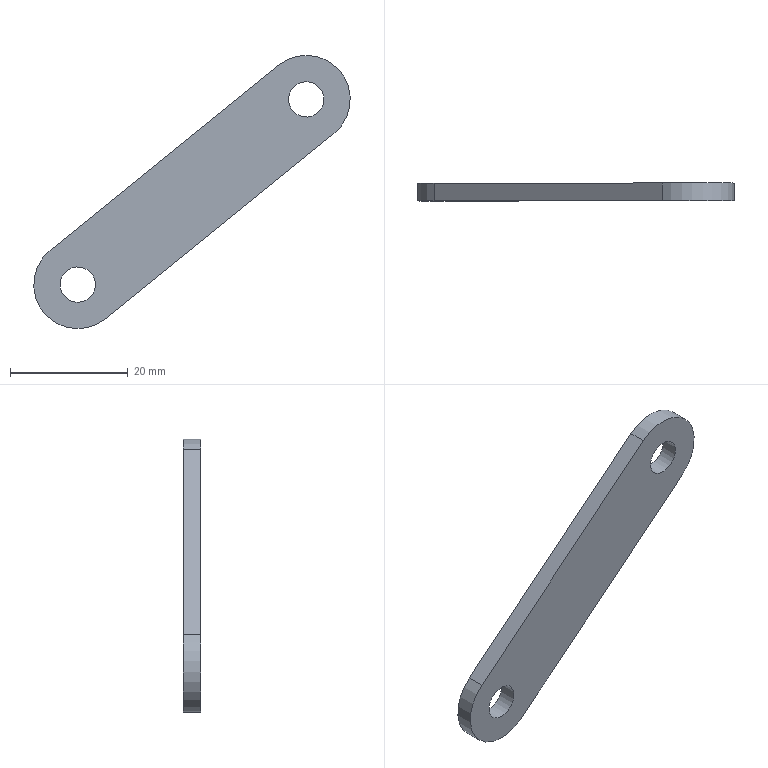Component | NX | LINK_1_3 | 1 solid | 8 faces | box 53.84 x 3 x 46.49 mm | volume 2610 mm3 | plane 4 | cylinder 4 | commonest cylinder face diameters 15 x2 6 x2
STEP:
#1=CARTESIAN_POINT('',(0.,0.,0.));
#2=DIRECTION('',(0.,0.,1.));
#3=DIRECTION('',(1.,0.,0.));
#4=AXIS2_PLACEMENT_3D('',#1,#2,#3);
#5=CARTESIAN_POINT('',(-181.438,80.,98.163));
#6=VERTEX_POINT('',#5);
#7=CARTESIAN_POINT('',(-220.277,80.,66.674));
#8=VERTEX_POINT('',#7);
#9=CARTESIAN_POINT('',(-181.438,80.,98.163));
#10=DIRECTION('',(-0.7768,0.,-0.6298));
#11=VECTOR('',#10,1.);
#12=LINE('',#9,#11);
#13=CARTESIAN_POINT('',(-181.438,77.,98.163));
#14=DIRECTION('',(0.6298,0.,-0.7768));
#15=DIRECTION('',(0.,1.,0.));
#16=AXIS2_PLACEMENT_3D('',#13,#14,#15);
#17=PLANE('',#16);
#18=CARTESIAN_POINT('',(3.,0.));
#19=DIRECTION('',(0.,-1.));
#20=VECTOR('',#19,1.);
#21=LINE('',#18,#20);
#22=(GEOMETRIC_REPRESENTATION_CONTEXT(2)PARAMETRIC_REPRESENTATION_CONTEXT()REPRESENTATION_CONTEXT('',''));
#23=DEFINITIONAL_REPRESENTATION('',(#21),#22);
#24=PCURVE('',#17,#23);
#25=CARTESIAN_POINT('',(-225.,80.,72.5));
#26=DIRECTION('',(0.,1.,0.));
#27=DIRECTION('',(-0.7768,0.,-0.6298));
#28=AXIS2_PLACEMENT_3D('',#25,#26,#27);
#29=PLANE('',#28);
#30=CARTESIAN_POINT('',(-50.,-7.5));
#31=DIRECTION('',(1.,0.));
#32=VECTOR('',#31,1.);
#33=LINE('',#30,#32);
#34=(GEOMETRIC_REPRESENTATION_CONTEXT(2)PARAMETRIC_REPRESENTATION_CONTEXT()REPRESENTATION_CONTEXT('',''));
#35=DEFINITIONAL_REPRESENTATION('',(#33),#34);
#36=PCURVE('',#29,#35);
#37=SURFACE_CURVE('',#12,(#24,#36),.PCURVE_S1.);
#38=EDGE_CURVE('',#6,#8,#37,.T.);
#39=ORIENTED_EDGE('',*,*,#38,.F.);
#40=CARTESIAN_POINT('',(-181.438,77.,98.163));
#41=VERTEX_POINT('',#40);
#42=CARTESIAN_POINT('',(-181.438,77.,98.163));
#43=DIRECTION('',(0.,1.,0.));
#44=VECTOR('',#43,1.);
#45=LINE('',#42,#44);
#46=CARTESIAN_POINT('',(0.,0.));
#47=DIRECTION('',(1.,0.));
#48=VECTOR('',#47,1.);
#49=LINE('',#46,#48);
#50=(GEOMETRIC_REPRESENTATION_CONTEXT(2)PARAMETRIC_REPRESENTATION_CONTEXT()REPRESENTATION_CONTEXT('',''));
#51=DEFINITIONAL_REPRESENTATION('',(#49),#50);
#52=PCURVE('',#17,#51);
#53=CARTESIAN_POINT('',(-186.161,77.,103.989));
#54=DIRECTION('',(0.,1.,0.));
#55=DIRECTION('',(-0.7768,0.,-0.6298));
#56=AXIS2_PLACEMENT_3D('',#53,#54,#55);
#57=CYLINDRICAL_SURFACE('',#56,7.5);
#58=CARTESIAN_POINT('',(4.712,0.));
#59=DIRECTION('',(0.,1.));
#60=VECTOR('',#59,1.);
#61=LINE('',#58,#60);
#62=(GEOMETRIC_REPRESENTATION_CONTEXT(2)PARAMETRIC_REPRESENTATION_CONTEXT()REPRESENTATION_CONTEXT('',''));
#63=DEFINITIONAL_REPRESENTATION('',(#61),#62);
#64=PCURVE('',#57,#63);
#65=SURFACE_CURVE('',#45,(#52,#64),.PCURVE_S1.);
#66=EDGE_CURVE('',#41,#6,#65,.T.);
#67=ORIENTED_EDGE('',*,*,#66,.F.);
#68=CARTESIAN_POINT('',(-220.277,77.,66.674));
#69=VERTEX_POINT('',#68);
#70=CARTESIAN_POINT('',(-181.438,77.,98.163));
#71=DIRECTION('',(-0.7768,0.,-0.6298));
#72=VECTOR('',#71,1.);
#73=LINE('',#70,#72);
#74=CARTESIAN_POINT('',(0.,0.));
#75=DIRECTION('',(0.,-1.));
#76=VECTOR('',#75,1.);
#77=LINE('',#74,#76);
#78=(GEOMETRIC_REPRESENTATION_CONTEXT(2)PARAMETRIC_REPRESENTATION_CONTEXT()REPRESENTATION_CONTEXT('',''));
#79=DEFINITIONAL_REPRESENTATION('',(#77),#78);
#80=PCURVE('',#17,#79);
#81=CARTESIAN_POINT('',(-225.,77.,72.5));
#82=DIRECTION('',(0.,1.,0.));
#83=DIRECTION('',(-0.7768,0.,-0.6298));
#84=AXIS2_PLACEMENT_3D('',#81,#82,#83);
#85=PLANE('',#84);
#86=CARTESIAN_POINT('',(-50.,-7.5));
#87=DIRECTION('',(1.,0.));
#88=VECTOR('',#87,1.);
#89=LINE('',#86,#88);
#90=(GEOMETRIC_REPRESENTATION_CONTEXT(2)PARAMETRIC_REPRESENTATION_CONTEXT()REPRESENTATION_CONTEXT('',''));
#91=DEFINITIONAL_REPRESENTATION('',(#89),#90);
#92=PCURVE('',#85,#91);
#93=SURFACE_CURVE('',#73,(#80,#92),.PCURVE_S1.);
#94=EDGE_CURVE('',#41,#69,#93,.T.);
#95=ORIENTED_EDGE('',*,*,#94,.T.);
#96=CARTESIAN_POINT('',(-220.277,77.,66.674));
#97=DIRECTION('',(0.,1.,0.));
#98=VECTOR('',#97,1.);
#99=LINE('',#96,#98);
#100=CARTESIAN_POINT('',(0.,-50.));
#101=DIRECTION('',(1.,0.));
#102=VECTOR('',#101,1.);
#103=LINE('',#100,#102);
#104=(GEOMETRIC_REPRESENTATION_CONTEXT(2)PARAMETRIC_REPRESENTATION_CONTEXT()REPRESENTATION_CONTEXT('',''));
#105=DEFINITIONAL_REPRESENTATION('',(#103),#104);
#106=PCURVE('',#17,#105);
#107=CARTESIAN_POINT('',(-225.,77.,72.5));
#108=DIRECTION('',(0.,1.,0.));
#109=DIRECTION('',(-0.7768,0.,-0.6298));
#110=AXIS2_PLACEMENT_3D('',#107,#108,#109);
#111=CYLINDRICAL_SURFACE('',#110,7.5);
#112=CARTESIAN_POINT('',(-1.571,0.));
#113=DIRECTION('',(0.,1.));
#114=VECTOR('',#113,1.);
#115=LINE('',#112,#114);
#116=(GEOMETRIC_REPRESENTATION_CONTEXT(2)PARAMETRIC_REPRESENTATION_CONTEXT()REPRESENTATION_CONTEXT('',''));
#117=DEFINITIONAL_REPRESENTATION('',(#115),#116);
#118=PCURVE('',#111,#117);
#119=SURFACE_CURVE('',#99,(#106,#118),.PCURVE_S1.);
#120=EDGE_CURVE('',#69,#8,#119,.T.);
#121=ORIENTED_EDGE('',*,*,#120,.T.);
#122=EDGE_LOOP('',(#39,#67,#95,#121));
#123=FACE_BOUND('',#122,.T.);
#124=ADVANCED_FACE('',(#123),#17,.T.);
#125=CARTESIAN_POINT('',(-229.723,80.,78.326));
#126=VERTEX_POINT('',#125);
#127=CARTESIAN_POINT('',(-225.,80.,72.5));
#128=DIRECTION('',(0.,1.,0.));
#129=DIRECTION('',(0.7768,0.,0.6298));
#130=AXIS2_PLACEMENT_3D('',#127,#128,#129);
#131=CIRCLE('',#130,7.5);
#132=CARTESIAN_POINT('',(-3.142,3.));
#133=DIRECTION('',(1.,0.));
#134=VECTOR('',#133,1.);
#135=LINE('',#132,#134);
#136=(GEOMETRIC_REPRESENTATION_CONTEXT(2)PARAMETRIC_REPRESENTATION_CONTEXT()REPRESENTATION_CONTEXT('',''));
#137=DEFINITIONAL_REPRESENTATION('',(#135),#136);
#138=PCURVE('',#111,#137);
#139=CARTESIAN_POINT('',(0.,0.));
#140=DIRECTION('',(-1.,0.));
#141=AXIS2_PLACEMENT_2D('',#139,#140);
#142=CIRCLE('',#141,7.5);
#143=(GEOMETRIC_REPRESENTATION_CONTEXT(2)PARAMETRIC_REPRESENTATION_CONTEXT()REPRESENTATION_CONTEXT('',''));
#144=DEFINITIONAL_REPRESENTATION('',(#142),#143);
#145=PCURVE('',#29,#144);
#146=SURFACE_CURVE('',#131,(#138,#145),.PCURVE_S1.);
#147=EDGE_CURVE('',#8,#126,#146,.T.);
#148=ORIENTED_EDGE('',*,*,#147,.F.);
#149=ORIENTED_EDGE('',*,*,#120,.F.);
#150=CARTESIAN_POINT('',(-229.723,77.,78.326));
#151=VERTEX_POINT('',#150);
#152=CARTESIAN_POINT('',(-225.,77.,72.5));
#153=DIRECTION('',(0.,1.,0.));
#154=DIRECTION('',(0.7768,0.,0.6298));
#155=AXIS2_PLACEMENT_3D('',#152,#153,#154);
#156=CIRCLE('',#155,7.5);
#157=CARTESIAN_POINT('',(-3.142,0.));
#158=DIRECTION('',(1.,0.));
#159=VECTOR('',#158,1.);
#160=LINE('',#157,#159);
#161=(GEOMETRIC_REPRESENTATION_CONTEXT(2)PARAMETRIC_REPRESENTATION_CONTEXT()REPRESENTATION_CONTEXT('',''));
#162=DEFINITIONAL_REPRESENTATION('',(#160),#161);
#163=PCURVE('',#111,#162);
#164=CARTESIAN_POINT('',(0.,0.));
#165=DIRECTION('',(-1.,0.));
#166=AXIS2_PLACEMENT_2D('',#164,#165);
#167=CIRCLE('',#166,7.5);
#168=(GEOMETRIC_REPRESENTATION_CONTEXT(2)PARAMETRIC_REPRESENTATION_CONTEXT()REPRESENTATION_CONTEXT('',''));
#169=DEFINITIONAL_REPRESENTATION('',(#167),#168);
#170=PCURVE('',#85,#169);
#171=SURFACE_CURVE('',#156,(#163,#170),.PCURVE_S1.);
#172=EDGE_CURVE('',#69,#151,#171,.T.);
#173=ORIENTED_EDGE('',*,*,#172,.T.);
#174=CARTESIAN_POINT('',(-229.723,77.,78.326));
#175=DIRECTION('',(0.,1.,0.));
#176=VECTOR('',#175,1.);
#177=LINE('',#174,#176);
#178=CARTESIAN_POINT('',(1.571,0.));
#179=DIRECTION('',(0.,1.));
#180=VECTOR('',#179,1.);
#181=LINE('',#178,#180);
#182=(GEOMETRIC_REPRESENTATION_CONTEXT(2)PARAMETRIC_REPRESENTATION_CONTEXT()REPRESENTATION_CONTEXT('',''));
#183=DEFINITIONAL_REPRESENTATION('',(#181),#182);
#184=PCURVE('',#111,#183);
#185=CARTESIAN_POINT('',(-229.723,77.,78.326));
#186=DIRECTION('',(-0.6298,0.,0.7768));
#187=DIRECTION('',(0.,-1.,0.));
#188=AXIS2_PLACEMENT_3D('',#185,#186,#187);
#189=PLANE('',#188);
#190=CARTESIAN_POINT('',(0.,0.));
#191=DIRECTION('',(-1.,0.));
#192=VECTOR('',#191,1.);
#193=LINE('',#190,#192);
#194=(GEOMETRIC_REPRESENTATION_CONTEXT(2)PARAMETRIC_REPRESENTATION_CONTEXT()REPRESENTATION_CONTEXT('',''));
#195=DEFINITIONAL_REPRESENTATION('',(#193),#194);
#196=PCURVE('',#189,#195);
#197=SURFACE_CURVE('',#177,(#184,#196),.PCURVE_S1.);
#198=EDGE_CURVE('',#151,#126,#197,.T.);
#199=ORIENTED_EDGE('',*,*,#198,.T.);
#200=EDGE_LOOP('',(#148,#149,#173,#199));
#201=FACE_BOUND('',#200,.T.);
#202=ADVANCED_FACE('',(#201),#111,.T.);
#203=CARTESIAN_POINT('',(-190.884,80.,109.815));
#204=VERTEX_POINT('',#203);
#205=CARTESIAN_POINT('',(-229.723,80.,78.326));
#206=DIRECTION('',(0.7768,0.,0.6298));
#207=VECTOR('',#206,1.);
#208=LINE('',#205,#207);
#209=CARTESIAN_POINT('',(-3.,0.));
#210=DIRECTION('',(0.,1.));
#211=VECTOR('',#210,1.);
#212=LINE('',#209,#211);
#213=(GEOMETRIC_REPRESENTATION_CONTEXT(2)PARAMETRIC_REPRESENTATION_CONTEXT()REPRESENTATION_CONTEXT('',''));
#214=DEFINITIONAL_REPRESENTATION('',(#212),#213);
#215=PCURVE('',#189,#214);
#216=CARTESIAN_POINT('',(0.,7.5));
#217=DIRECTION('',(-1.,0.));
#218=VECTOR('',#217,1.);
#219=LINE('',#216,#218);
#220=(GEOMETRIC_REPRESENTATION_CONTEXT(2)PARAMETRIC_REPRESENTATION_CONTEXT()REPRESENTATION_CONTEXT('',''));
#221=DEFINITIONAL_REPRESENTATION('',(#219),#220);
#222=PCURVE('',#29,#221);
#223=SURFACE_CURVE('',#208,(#215,#222),.PCURVE_S1.);
#224=EDGE_CURVE('',#126,#204,#223,.T.);
#225=ORIENTED_EDGE('',*,*,#224,.F.);
#226=ORIENTED_EDGE('',*,*,#198,.F.);
#227=CARTESIAN_POINT('',(-190.884,77.,109.815));
#228=VERTEX_POINT('',#227);
#229=CARTESIAN_POINT('',(-229.723,77.,78.326));
#230=DIRECTION('',(0.7768,0.,0.6298));
#231=VECTOR('',#230,1.);
#232=LINE('',#229,#231);
#233=CARTESIAN_POINT('',(0.,0.));
#234=DIRECTION('',(0.,1.));
#235=VECTOR('',#234,1.);
#236=LINE('',#233,#235);
#237=(GEOMETRIC_REPRESENTATION_CONTEXT(2)PARAMETRIC_REPRESENTATION_CONTEXT()REPRESENTATION_CONTEXT('',''));
#238=DEFINITIONAL_REPRESENTATION('',(#236),#237);
#239=PCURVE('',#189,#238);
#240=CARTESIAN_POINT('',(0.,7.5));
#241=DIRECTION('',(-1.,0.));
#242=VECTOR('',#241,1.);
#243=LINE('',#240,#242);
#244=(GEOMETRIC_REPRESENTATION_CONTEXT(2)PARAMETRIC_REPRESENTATION_CONTEXT()REPRESENTATION_CONTEXT('',''));
#245=DEFINITIONAL_REPRESENTATION('',(#243),#244);
#246=PCURVE('',#85,#245);
#247=SURFACE_CURVE('',#232,(#239,#246),.PCURVE_S1.);
#248=EDGE_CURVE('',#151,#228,#247,.T.);
#249=ORIENTED_EDGE('',*,*,#248,.T.);
#250=CARTESIAN_POINT('',(-190.884,77.,109.815));
#251=DIRECTION('',(0.,1.,0.));
#252=VECTOR('',#251,1.);
#253=LINE('',#250,#252);
#254=CARTESIAN_POINT('',(0.,50.));
#255=DIRECTION('',(-1.,0.));
#256=VECTOR('',#255,1.);
#257=LINE('',#254,#256);
#258=(GEOMETRIC_REPRESENTATION_CONTEXT(2)PARAMETRIC_REPRESENTATION_CONTEXT()REPRESENTATION_CONTEXT('',''));
#259=DEFINITIONAL_REPRESENTATION('',(#257),#258);
#260=PCURVE('',#189,#259);
#261=CARTESIAN_POINT('',(1.571,0.));
#262=DIRECTION('',(0.,1.));
#263=VECTOR('',#262,1.);
#264=LINE('',#261,#263);
#265=(GEOMETRIC_REPRESENTATION_CONTEXT(2)PARAMETRIC_REPRESENTATION_CONTEXT()REPRESENTATION_CONTEXT('',''));
#266=DEFINITIONAL_REPRESENTATION('',(#264),#265);
#267=PCURVE('',#57,#266);
#268=SURFACE_CURVE('',#253,(#260,#267),.PCURVE_S1.);
#269=EDGE_CURVE('',#228,#204,#268,.T.);
#270=ORIENTED_EDGE('',*,*,#269,.T.);
#271=EDGE_LOOP('',(#225,#226,#249,#270));
#272=FACE_BOUND('',#271,.T.);
#273=ADVANCED_FACE('',(#272),#189,.T.);
#274=CARTESIAN_POINT('',(-188.491,77.,102.099));
#275=VERTEX_POINT('',#274);
#276=CARTESIAN_POINT('',(-186.161,77.,103.989));
#277=DIRECTION('',(0.,-1.,0.));
#278=DIRECTION('',(-0.7768,0.,-0.6298));
#279=AXIS2_PLACEMENT_3D('',#276,#277,#278);
#280=CIRCLE('',#279,3.);
#281=CARTESIAN_POINT('',(-186.161,77.,103.989));
#282=DIRECTION('',(0.,1.,0.));
#283=DIRECTION('',(-0.7768,0.,-0.6298));
#284=AXIS2_PLACEMENT_3D('',#281,#282,#283);
#285=CYLINDRICAL_SURFACE('',#284,3.);
#286=CARTESIAN_POINT('',(6.283,0.));
#287=DIRECTION('',(-1.,0.));
#288=VECTOR('',#287,1.);
#289=LINE('',#286,#288);
#290=(GEOMETRIC_REPRESENTATION_CONTEXT(2)PARAMETRIC_REPRESENTATION_CONTEXT()REPRESENTATION_CONTEXT('',''));
#291=DEFINITIONAL_REPRESENTATION('',(#289),#290);
#292=PCURVE('',#285,#291);
#293=CARTESIAN_POINT('',(-47.,-0.));
#294=CARTESIAN_POINT('',(-47.,-5.196));
#295=CARTESIAN_POINT('',(-51.5,-2.598));
#296=CARTESIAN_POINT('',(-56.,-0.));
#297=CARTESIAN_POINT('',(-51.5,2.598));
#298=CARTESIAN_POINT('',(-47.,5.196));
#299=CARTESIAN_POINT('',(-47.,-0.));
#300=(BOUNDED_CURVE()B_SPLINE_CURVE(2,(#293,#294,#295,#296,#297,#298,#299),.UNSPECIFIED.,.T.,.F.)B_SPLINE_CURVE_WITH_KNOTS((1,2,2,2,2,1),(-2.094,0.,2.094,4.189,6.283,8.378),.UNSPECIFIED.)CURVE()GEOMETRIC_REPRESENTATION_ITEM()RATIONAL_B_SPLINE_CURVE((1.,0.5,1.,0.5,1.,0.5,1.))REPRESENTATION_ITEM(''));
#301=(GEOMETRIC_REPRESENTATION_CONTEXT(2)PARAMETRIC_REPRESENTATION_CONTEXT()REPRESENTATION_CONTEXT('',''));
#302=DEFINITIONAL_REPRESENTATION('',(#300),#301);
#303=PCURVE('',#85,#302);
#304=SURFACE_CURVE('',#280,(#292,#303),.PCURVE_S1.);
#305=EDGE_CURVE('',#275,#275,#304,.T.);
#306=ORIENTED_EDGE('',*,*,#305,.F.);
#307=CARTESIAN_POINT('',(-188.491,80.,102.099));
#308=VERTEX_POINT('',#307);
#309=CARTESIAN_POINT('',(-188.491,77.,102.099));
#310=CARTESIAN_POINT('',(-188.491,80.,102.099));
#311=B_SPLINE_CURVE_WITH_KNOTS('',1,(#309,#310),.UNSPECIFIED.,.F.,.F.,(2,2),(0.,3.),.PIECEWISE_BEZIER_KNOTS.);
#312=CARTESIAN_POINT('',(6.283,0.));
#313=DIRECTION('',(0.,1.));
#314=VECTOR('',#313,1.);
#315=LINE('',#312,#314);
#316=(GEOMETRIC_REPRESENTATION_CONTEXT(2)PARAMETRIC_REPRESENTATION_CONTEXT()REPRESENTATION_CONTEXT('',''));
#317=DEFINITIONAL_REPRESENTATION('',(#315),#316);
#318=PCURVE('',#285,#317);
#319=CARTESIAN_POINT('',(0.,0.));
#320=DIRECTION('',(0.,1.));
#321=VECTOR('',#320,1.);
#322=LINE('',#319,#321);
#323=(GEOMETRIC_REPRESENTATION_CONTEXT(2)PARAMETRIC_REPRESENTATION_CONTEXT()REPRESENTATION_CONTEXT('',''));
#324=DEFINITIONAL_REPRESENTATION('',(#322),#323);
#325=PCURVE('',#285,#324);
#326=SEAM_CURVE('',#311,(#318,#325),.PCURVE_S1.);
#327=EDGE_CURVE('',#275,#308,#326,.T.);
#328=ORIENTED_EDGE('',*,*,#327,.T.);
#329=CARTESIAN_POINT('',(-186.161,80.,103.989));
#330=DIRECTION('',(0.,-1.,0.));
#331=DIRECTION('',(-0.7768,0.,-0.6298));
#332=AXIS2_PLACEMENT_3D('',#329,#330,#331);
#333=CIRCLE('',#332,3.);
#334=CARTESIAN_POINT('',(6.283,3.));
#335=DIRECTION('',(-1.,0.));
#336=VECTOR('',#335,1.);
#337=LINE('',#334,#336);
#338=(GEOMETRIC_REPRESENTATION_CONTEXT(2)PARAMETRIC_REPRESENTATION_CONTEXT()REPRESENTATION_CONTEXT('',''));
#339=DEFINITIONAL_REPRESENTATION('',(#337),#338);
#340=PCURVE('',#285,#339);
#341=CARTESIAN_POINT('',(-47.,-0.));
#342=CARTESIAN_POINT('',(-47.,-5.196));
#343=CARTESIAN_POINT('',(-51.5,-2.598));
#344=CARTESIAN_POINT('',(-56.,-0.));
#345=CARTESIAN_POINT('',(-51.5,2.598));
#346=CARTESIAN_POINT('',(-47.,5.196));
#347=CARTESIAN_POINT('',(-47.,-0.));
#348=(BOUNDED_CURVE()B_SPLINE_CURVE(2,(#341,#342,#343,#344,#345,#346,#347),.UNSPECIFIED.,.T.,.F.)B_SPLINE_CURVE_WITH_KNOTS((1,2,2,2,2,1),(-2.094,0.,2.094,4.189,6.283,8.378),.UNSPECIFIED.)CURVE()GEOMETRIC_REPRESENTATION_ITEM()RATIONAL_B_SPLINE_CURVE((1.,0.5,1.,0.5,1.,0.5,1.))REPRESENTATION_ITEM(''));
#349=(GEOMETRIC_REPRESENTATION_CONTEXT(2)PARAMETRIC_REPRESENTATION_CONTEXT()REPRESENTATION_CONTEXT('',''));
#350=DEFINITIONAL_REPRESENTATION('',(#348),#349);
#351=PCURVE('',#29,#350);
#352=SURFACE_CURVE('',#333,(#340,#351),.PCURVE_S1.);
#353=EDGE_CURVE('',#308,#308,#352,.T.);
#354=ORIENTED_EDGE('',*,*,#353,.T.);
#355=ORIENTED_EDGE('',*,*,#327,.F.);
#356=EDGE_LOOP('',(#306,#328,#354,#355));
#357=FACE_BOUND('',#356,.F.);
#358=ADVANCED_FACE('',(#357),#285,.F.);
#359=CARTESIAN_POINT('',(-186.161,80.,103.989));
#360=DIRECTION('',(0.,1.,0.));
#361=DIRECTION('',(-0.7768,0.,-0.6298));
#362=AXIS2_PLACEMENT_3D('',#359,#360,#361);
#363=CIRCLE('',#362,7.5);
#364=CARTESIAN_POINT('',(0.,3.));
#365=DIRECTION('',(1.,0.));
#366=VECTOR('',#365,1.);
#367=LINE('',#364,#366);
#368=(GEOMETRIC_REPRESENTATION_CONTEXT(2)PARAMETRIC_REPRESENTATION_CONTEXT()REPRESENTATION_CONTEXT('',''));
#369=DEFINITIONAL_REPRESENTATION('',(#367),#368);
#370=PCURVE('',#57,#369);
#371=CARTESIAN_POINT('',(-50.,-0.));
#372=DIRECTION('',(1.,-0.));
#373=AXIS2_PLACEMENT_2D('',#371,#372);
#374=CIRCLE('',#373,7.5);
#375=(GEOMETRIC_REPRESENTATION_CONTEXT(2)PARAMETRIC_REPRESENTATION_CONTEXT()REPRESENTATION_CONTEXT('',''));
#376=DEFINITIONAL_REPRESENTATION('',(#374),#375);
#377=PCURVE('',#29,#376);
#378=SURFACE_CURVE('',#363,(#370,#377),.PCURVE_S1.);
#379=EDGE_CURVE('',#204,#6,#378,.T.);
#380=ORIENTED_EDGE('',*,*,#379,.F.);
#381=ORIENTED_EDGE('',*,*,#269,.F.);
#382=CARTESIAN_POINT('',(-186.161,77.,103.989));
#383=DIRECTION('',(0.,1.,0.));
#384=DIRECTION('',(-0.7768,0.,-0.6298));
#385=AXIS2_PLACEMENT_3D('',#382,#383,#384);
#386=CIRCLE('',#385,7.5);
#387=CARTESIAN_POINT('',(0.,0.));
#388=DIRECTION('',(1.,0.));
#389=VECTOR('',#388,1.);
#390=LINE('',#387,#389);
#391=(GEOMETRIC_REPRESENTATION_CONTEXT(2)PARAMETRIC_REPRESENTATION_CONTEXT()REPRESENTATION_CONTEXT('',''));
#392=DEFINITIONAL_REPRESENTATION('',(#390),#391);
#393=PCURVE('',#57,#392);
#394=CARTESIAN_POINT('',(-50.,-0.));
#395=DIRECTION('',(1.,-0.));
#396=AXIS2_PLACEMENT_2D('',#394,#395);
#397=CIRCLE('',#396,7.5);
#398=(GEOMETRIC_REPRESENTATION_CONTEXT(2)PARAMETRIC_REPRESENTATION_CONTEXT()REPRESENTATION_CONTEXT('',''));
#399=DEFINITIONAL_REPRESENTATION('',(#397),#398);
#400=PCURVE('',#85,#399);
#401=SURFACE_CURVE('',#386,(#393,#400),.PCURVE_S1.);
#402=EDGE_CURVE('',#228,#41,#401,.T.);
#403=ORIENTED_EDGE('',*,*,#402,.T.);
#404=ORIENTED_EDGE('',*,*,#66,.T.);
#405=EDGE_LOOP('',(#380,#381,#403,#404));
#406=FACE_BOUND('',#405,.T.);
#407=ADVANCED_FACE('',(#406),#57,.T.);
#408=CARTESIAN_POINT('',(-222.67,77.,74.389));
#409=VERTEX_POINT('',#408);
#410=CARTESIAN_POINT('',(-225.,77.,72.5));
#411=DIRECTION('',(0.,1.,0.));
#412=DIRECTION('',(0.7768,0.,0.6298));
#413=AXIS2_PLACEMENT_3D('',#410,#411,#412);
#414=CIRCLE('',#413,3.);
#415=CARTESIAN_POINT('',(-225.,77.,72.5));
#416=DIRECTION('',(0.,1.,0.));
#417=DIRECTION('',(-0.7768,0.,-0.6298));
#418=AXIS2_PLACEMENT_3D('',#415,#416,#417);
#419=CYLINDRICAL_SURFACE('',#418,3.);
#420=CARTESIAN_POINT('',(3.142,0.));
#421=DIRECTION('',(1.,0.));
#422=VECTOR('',#421,1.);
#423=LINE('',#420,#422);
#424=(GEOMETRIC_REPRESENTATION_CONTEXT(2)PARAMETRIC_REPRESENTATION_CONTEXT()REPRESENTATION_CONTEXT('',''));
#425=DEFINITIONAL_REPRESENTATION('',(#423),#424);
#426=PCURVE('',#419,#425);
#427=CARTESIAN_POINT('',(0.,0.));
#428=DIRECTION('',(-1.,0.));
#429=AXIS2_PLACEMENT_2D('',#427,#428);
#430=CIRCLE('',#429,3.);
#431=(GEOMETRIC_REPRESENTATION_CONTEXT(2)PARAMETRIC_REPRESENTATION_CONTEXT()REPRESENTATION_CONTEXT('',''));
#432=DEFINITIONAL_REPRESENTATION('',(#430),#431);
#433=PCURVE('',#85,#432);
#434=SURFACE_CURVE('',#414,(#426,#433),.PCURVE_S1.);
#435=EDGE_CURVE('',#409,#409,#434,.T.);
#436=ORIENTED_EDGE('',*,*,#435,.T.);
#437=CARTESIAN_POINT('',(-222.67,80.,74.389));
#438=VERTEX_POINT('',#437);
#439=CARTESIAN_POINT('',(-222.67,77.,74.389));
#440=CARTESIAN_POINT('',(-222.67,80.,74.389));
#441=B_SPLINE_CURVE_WITH_KNOTS('',1,(#439,#440),.UNSPECIFIED.,.F.,.F.,(2,2),(0.,3.),.PIECEWISE_BEZIER_KNOTS.);
#442=CARTESIAN_POINT('',(9.425,0.));
#443=DIRECTION('',(0.,1.));
#444=VECTOR('',#443,1.);
#445=LINE('',#442,#444);
#446=(GEOMETRIC_REPRESENTATION_CONTEXT(2)PARAMETRIC_REPRESENTATION_CONTEXT()REPRESENTATION_CONTEXT('',''));
#447=DEFINITIONAL_REPRESENTATION('',(#445),#446);
#448=PCURVE('',#419,#447);
#449=CARTESIAN_POINT('',(3.142,0.));
#450=DIRECTION('',(0.,1.));
#451=VECTOR('',#450,1.);
#452=LINE('',#449,#451);
#453=(GEOMETRIC_REPRESENTATION_CONTEXT(2)PARAMETRIC_REPRESENTATION_CONTEXT()REPRESENTATION_CONTEXT('',''));
#454=DEFINITIONAL_REPRESENTATION('',(#452),#453);
#455=PCURVE('',#419,#454);
#456=SEAM_CURVE('',#441,(#448,#455),.PCURVE_S1.);
#457=EDGE_CURVE('',#409,#438,#456,.T.);
#458=ORIENTED_EDGE('',*,*,#457,.T.);
#459=CARTESIAN_POINT('',(-225.,80.,72.5));
#460=DIRECTION('',(0.,1.,0.));
#461=DIRECTION('',(0.7768,0.,0.6298));
#462=AXIS2_PLACEMENT_3D('',#459,#460,#461);
#463=CIRCLE('',#462,3.);
#464=CARTESIAN_POINT('',(3.142,3.));
#465=DIRECTION('',(1.,0.));
#466=VECTOR('',#465,1.);
#467=LINE('',#464,#466);
#468=(GEOMETRIC_REPRESENTATION_CONTEXT(2)PARAMETRIC_REPRESENTATION_CONTEXT()REPRESENTATION_CONTEXT('',''));
#469=DEFINITIONAL_REPRESENTATION('',(#467),#468);
#470=PCURVE('',#419,#469);
#471=CARTESIAN_POINT('',(0.,0.));
#472=DIRECTION('',(-1.,0.));
#473=AXIS2_PLACEMENT_2D('',#471,#472);
#474=CIRCLE('',#473,3.);
#475=(GEOMETRIC_REPRESENTATION_CONTEXT(2)PARAMETRIC_REPRESENTATION_CONTEXT()REPRESENTATION_CONTEXT('',''));
#476=DEFINITIONAL_REPRESENTATION('',(#474),#475);
#477=PCURVE('',#29,#476);
#478=SURFACE_CURVE('',#463,(#470,#477),.PCURVE_S1.);
#479=EDGE_CURVE('',#438,#438,#478,.T.);
#480=ORIENTED_EDGE('',*,*,#479,.F.);
#481=ORIENTED_EDGE('',*,*,#457,.F.);
#482=EDGE_LOOP('',(#436,#458,#480,#481));
#483=FACE_BOUND('',#482,.F.);
#484=ADVANCED_FACE('',(#483),#419,.F.);
#485=ORIENTED_EDGE('',*,*,#94,.F.);
#486=ORIENTED_EDGE('',*,*,#402,.F.);
#487=ORIENTED_EDGE('',*,*,#248,.F.);
#488=ORIENTED_EDGE('',*,*,#172,.F.);
#489=EDGE_LOOP('',(#485,#486,#487,#488));
#490=FACE_BOUND('',#489,.T.);
#491=ORIENTED_EDGE('',*,*,#305,.F.);
#492=EDGE_LOOP('',(#491));
#493=FACE_BOUND('',#492,.T.);
#494=ORIENTED_EDGE('',*,*,#435,.T.);
#495=EDGE_LOOP('',(#494));
#496=FACE_BOUND('',#495,.T.);
#497=ADVANCED_FACE('',(#490,#493,#496),#85,.F.);
#498=ORIENTED_EDGE('',*,*,#38,.T.);
#499=ORIENTED_EDGE('',*,*,#147,.T.);
#500=ORIENTED_EDGE('',*,*,#224,.T.);
#501=ORIENTED_EDGE('',*,*,#379,.T.);
#502=EDGE_LOOP('',(#498,#499,#500,#501));
#503=FACE_BOUND('',#502,.T.);
#504=ORIENTED_EDGE('',*,*,#353,.T.);
#505=EDGE_LOOP('',(#504));
#506=FACE_BOUND('',#505,.T.);
#507=ORIENTED_EDGE('',*,*,#479,.F.);
#508=EDGE_LOOP('',(#507));
#509=FACE_BOUND('',#508,.T.);
#510=ADVANCED_FACE('',(#503,#506,#509),#29,.T.);
#511=CLOSED_SHELL('',(#124,#202,#273,#358,#407,#484,#497,#510));
#512=MANIFOLD_SOLID_BREP('',#511);
#513=(LENGTH_UNIT()NAMED_UNIT(*)SI_UNIT(.MILLI.,.METRE.));
#514=UNCERTAINTY_MEASURE_WITH_UNIT(LENGTH_MEASURE(0.000002),#513,'','');
#515=(NAMED_UNIT(*)PLANE_ANGLE_UNIT()SI_UNIT($,.RADIAN.));
#516=(NAMED_UNIT(*)SI_UNIT($,.STERADIAN.)SOLID_ANGLE_UNIT());
#517=(GEOMETRIC_REPRESENTATION_CONTEXT(3)GLOBAL_UNCERTAINTY_ASSIGNED_CONTEXT((#514))GLOBAL_UNIT_ASSIGNED_CONTEXT((#513,#515,#516))REPRESENTATION_CONTEXT('',''));
#518=ADVANCED_BREP_SHAPE_REPRESENTATION('',(#4,#512),#517);